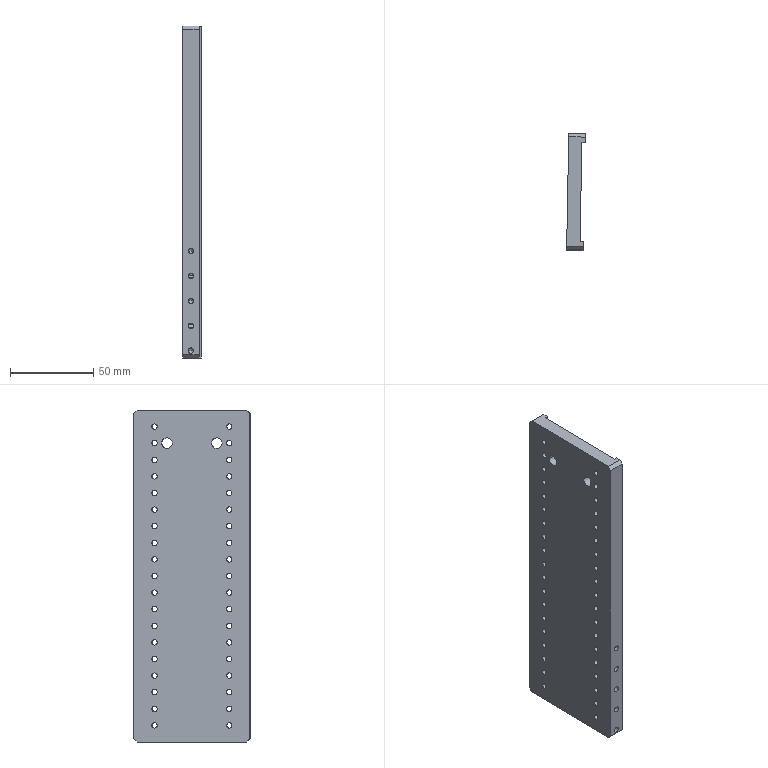Component | SolidWorks | DM17A08-02-033-2 | 1 solid | 130 faces | box 11.31 x 70.18 x 200 mm | volume 111817 mm3 | cylinder 100 | cone 16 | plane 14 | commonest cylinder face diameters 3.3 x96 6.4 x4 | material 6061 Alloy
build123d program:
from build123d import *

# Parameters (mm, degrees)
SKETCH1_W                  = 70
SKETCH1_H                  = 200
BOSS_EXTRUDE1_DEPTH        = 10
SKETCH2_W                  = 60
SKETCH2_H                  = 200
CUT_EXTRUDE1_DEPTH         = 2
CHAMFER1_SIZE              = 2
M4_TAPPED_HOLE1_D          = 3.3
LPATTERN1_COUNT            = 19
LPATTERN1_PITCH            = 10
M4_TAPPED_HOLE2_AT_2_COUNT = 2
M4_TAPPED_HOLE2_AT_2_PITCH = 15
M4_TAPPED_HOLE2_AT_3_COUNT = 2
M4_TAPPED_HOLE2_AT_3_PITCH = 30
M4_TAPPED_HOLE2_AT_4_COUNT = 2
M4_TAPPED_HOLE2_AT_4_PITCH = 45
M6_CLEARANCE_HOLE1_D       = 6.4


with BuildPart() as part:
    # Sketch1 → Boss-Extrude1 (new body)
    with BuildSketch(Plane.XY):
        Rectangle(SKETCH1_W, SKETCH1_H)
    extrude(amount=BOSS_EXTRUDE1_DEPTH)

    # Sketch2 → Cut-Extrude1 (cut)
    with BuildSketch(Plane.XY.offset(10)):
        Rectangle(SKETCH2_W, SKETCH2_H)
    extrude(amount=-CUT_EXTRUDE1_DEPTH, mode=Mode.SUBTRACT)

    # Chamfer1
    chamfer1_edges = [part.edges().sort_by_distance(p)[0] for p in [
        (35, -100, 5),
        (-35, -100, 5),
        (-35, 100, 5),
        (35, 100, 5),
    ]]
    chamfer(chamfer1_edges, length=CHAMFER1_SIZE)

    # M4 Tapped Hole1 (through all)
    with Locations(Plane.XY.offset(8)):
        with Locations((-22.5, 90), (22.5, 90)):
            m4_tapped_hole1 = Hole(M4_TAPPED_HOLE1_D / 2)

    # LPattern1: M4 Tapped Hole1 ×19
    with Locations(*[(0, -i * LPATTERN1_PITCH, 0) for i in range(1, LPATTERN1_COUNT)]):
        add(m4_tapped_hole1, mode=Mode.SUBTRACT)

    # Sketch7 → M4 Tapped Hole2 (revolve, cut)
    with BuildSketch(Plane(origin=(35, -35.571, 5), x_dir=(0, 0, -1), z_dir=(0, 1, 0))):
        Polygon((0, 0), (0, 12.491), (1.65, 11.5), (1.65, 0), align=None)
    m4_tapped_hole2 = revolve(axis=Axis((41.35, -35.571, 5), (-1, 0, 0)), mode=Mode.SUBTRACT)

    # M4 Tapped Hole2 at 2: M4 Tapped Hole2 ×2
    with Locations(*[(0, -i * M4_TAPPED_HOLE2_AT_2_PITCH, 0) for i in range(1, M4_TAPPED_HOLE2_AT_2_COUNT)]):
        add(m4_tapped_hole2, mode=Mode.SUBTRACT)

    # M4 Tapped Hole2 at 3: M4 Tapped Hole2 ×2
    with Locations(*[(0, -i * M4_TAPPED_HOLE2_AT_3_PITCH, 0) for i in range(1, M4_TAPPED_HOLE2_AT_3_COUNT)]):
        add(m4_tapped_hole2, mode=Mode.SUBTRACT)

    # M4 Tapped Hole2 at 4: M4 Tapped Hole2 ×2
    with Locations(*[(0, -i * M4_TAPPED_HOLE2_AT_4_PITCH, 0) for i in range(1, M4_TAPPED_HOLE2_AT_4_COUNT)]):
        add(m4_tapped_hole2, mode=Mode.SUBTRACT)

    # Sketch9 → M4 Tapped Hole3 (revolve, cut)
    with BuildSketch(Plane(origin=(35, -95.571, 5), x_dir=(0, 0, -1), z_dir=(0, 1, 0))):
        Polygon((0, 0), (0, 12.491), (1.65, 11.5), (1.65, 0), align=None)
    m4_tapped_hole3 = revolve(axis=Axis((41.35, -95.571, 5), (-1, 0, 0)), mode=Mode.SUBTRACT)

    # M6 Clearance Hole1 (through all)
    with Locations(Plane.XY.offset(8)):
        with Locations((-15, 80), (15, 80)):
            Hole(M6_CLEARANCE_HOLE1_D / 2)

    # Mirror1: M4 Tapped Hole2, M4 Tapped Hole3 across plane
    add(m4_tapped_hole2.mirror(Plane(origin=(0, 0, 0), x_dir=(0, 0, 1), z_dir=(1, 0, 0))), mode=Mode.SUBTRACT)
    add(m4_tapped_hole3.mirror(Plane(origin=(0, 0, 0), x_dir=(0, 0, 1), z_dir=(1, 0, 0))), mode=Mode.SUBTRACT)

    # Mirror1 copy 1 sketch → Mirror1 copy 1 (revolve, cut)
    with BuildSketch(Plane(origin=(-35, -50.571, 5), x_dir=(0, 0, -1), z_dir=(0, 1, 0))):
        Polygon((0, 0), (0, -12.491), (1.65, -11.5), (1.65, 0), align=None)
    revolve(axis=Axis((-41.35, -50.571, 5), (-1, 0, 0)), mode=Mode.SUBTRACT)

    # Mirror1 copy 2 sketch → Mirror1 copy 2 (revolve, cut)
    with BuildSketch(Plane(origin=(-35, -65.571, 5), x_dir=(0, 0, -1), z_dir=(0, 1, 0))):
        Polygon((0, 0), (0, -12.491), (1.65, -11.5), (1.65, 0), align=None)
    revolve(axis=Axis((-41.35, -65.571, 5), (-1, 0, 0)), mode=Mode.SUBTRACT)

    # Mirror1 copy 3 sketch → Mirror1 copy 3 (revolve, cut)
    with BuildSketch(Plane(origin=(-35, -80.571, 5), x_dir=(0, 0, -1), z_dir=(0, 1, 0))):
        Polygon((0, 0), (0, -12.491), (1.65, -11.5), (1.65, 0), align=None)
    revolve(axis=Axis((-41.35, -80.571, 5), (-1, 0, 0)), mode=Mode.SUBTRACT)


solid = part.part

# Placed as in the assembly
solid = solid.moved(Location((506.37, 441.829, 1115.565), (90, 88.927, 0)))